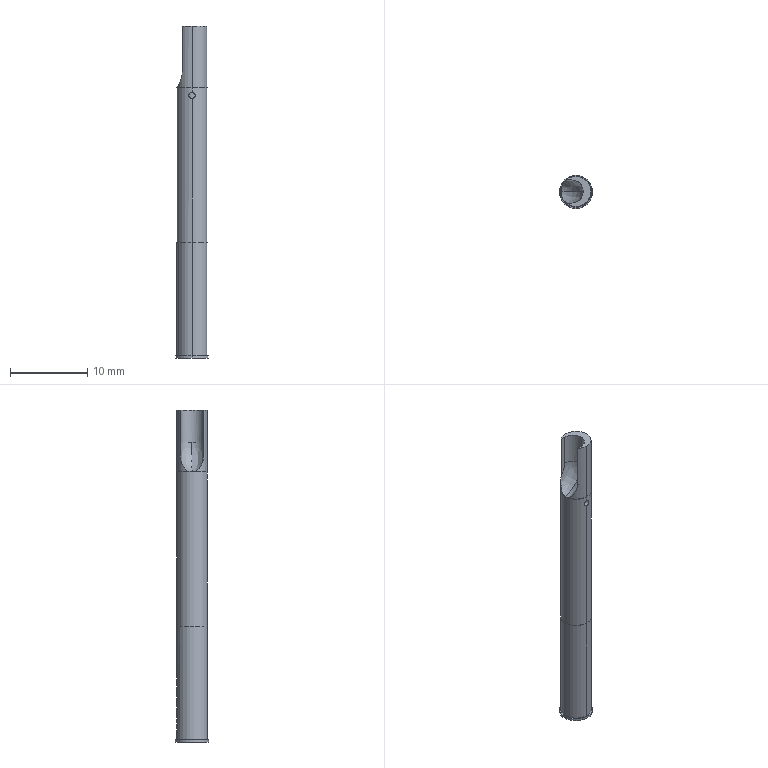Component | SolidWorks | 170423A4-INGUN HSS150-1_170423A4-INGUN_KS-150_30_M3_0-1 | 1 solid | 96 faces | box 4.3 x 4.3 x 43 mm | volume 166 mm3 | plane 48 | spline 24 | cylinder 24 | commonest cylinder face diameters 3.9 x8 4 x6 3.5 x2 3.96 x2 0.8 x2 4.3 x2 2.387 x1 3 x1